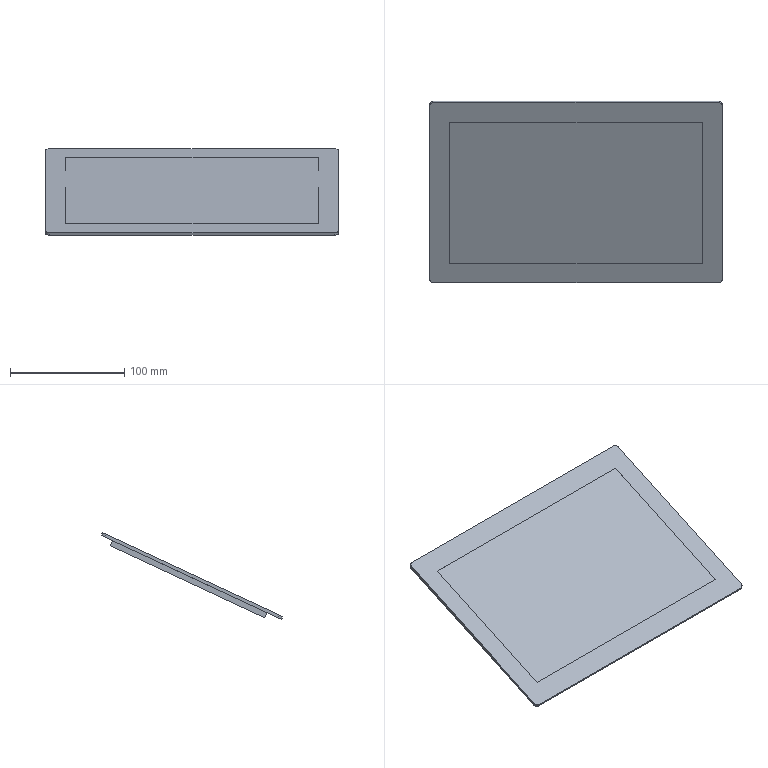Component | SolidWorks | 10.1InchScreen-1 | 1 solid | 20 faces | box 256.55 x 159.21 x 76.01 mm | volume 282503 mm3 | plane 16 | cylinder 4 | commonest cylinder face diameters 7 x4
build123d program:
from build123d import *

# Parameters (mm, degrees)
BOSS_EXTRUDE1_DEPTH = 2.5
SKETCH2_W           = 228.95
SKETCH2_H           = 149.3
BOSS_EXTRUDE2_DEPTH = 5
SKETCH3_W           = 221.1
SKETCH3_H           = 136.4
CUT_EXTRUDE1_DEPTH  = 0.01


with BuildPart() as part:
    # Sketch1 → Boss-Extrude1 (new body)
    with BuildSketch(Plane.XY):
        with BuildLine():
            Line((-124.775, -87.25), (124.775, -87.25))
            ThreePointArc((124.775, -87.25), (127.25, -86.225), (128.275, -83.75))
            Line((128.275, -83.75), (128.275, 83.75))
            ThreePointArc((128.275, 83.75), (127.25, 86.225), (124.775, 87.25))
            Line((124.775, 87.25), (-124.775, 87.25))
            ThreePointArc((-124.775, 87.25), (-127.25, 86.225), (-128.275, 83.75))
            Line((-128.275, 83.75), (-128.275, -83.75))
            ThreePointArc((-128.275, -83.75), (-127.25, -86.225), (-124.775, -87.25))
        make_face()
    extrude(amount=BOSS_EXTRUDE1_DEPTH)

    # Sketch2 → Boss-Extrude2 (add)
    with BuildSketch(Plane(origin=(0, 0, 0), x_dir=(-1, 0, 0), z_dir=(0, 0, -1))):
        with Locations((0, 1.4)):
            Rectangle(SKETCH2_W, SKETCH2_H)
    extrude(amount=BOSS_EXTRUDE2_DEPTH)

    # Sketch3 → Cut-Extrude1 (cut)
    with BuildSketch(Plane.XY.offset(2.5)):
        Rectangle(SKETCH3_W, SKETCH3_H)
    extrude(amount=-CUT_EXTRUDE1_DEPTH, mode=Mode.SUBTRACT)


solid = part.part

# Placed as in the assembly
solid = solid.moved(Location((1137.911, 1551.916, 2465.753), (25, 0, 0)))
STEP:
#1=CARTESIAN_POINT('',(49.712,57.986,95.625));
#2=VERTEX_POINT('',#1);
#3=CARTESIAN_POINT('',(49.85,58.111,95.683));
#4=VERTEX_POINT('',#3);
#5=CARTESIAN_POINT('',(49.712,58.111,95.683));
#6=DIRECTION('',(0.,-0.4226,0.9063));
#7=DIRECTION('',(1.,0.,0.));
#8=AXIS2_PLACEMENT_3D('',#5,#6,#7);
#9=CIRCLE('',#8,0.1378);
#10=EDGE_CURVE('',#2,#4,#9,.T.);
#11=ORIENTED_EDGE('',*,*,#10,.F.);
#12=CARTESIAN_POINT('',(39.887,57.986,95.625));
#13=VERTEX_POINT('',#12);
#14=CARTESIAN_POINT('',(39.887,57.986,95.625));
#15=DIRECTION('',(1.,0.,-0.));
#16=VECTOR('',#15,39.37);
#17=LINE('',#14,#16);
#18=EDGE_CURVE('',#13,#2,#17,.T.);
#19=ORIENTED_EDGE('',*,*,#18,.F.);
#20=CARTESIAN_POINT('',(39.749,58.111,95.683));
#21=VERTEX_POINT('',#20);
#22=CARTESIAN_POINT('',(39.887,58.111,95.683));
#23=DIRECTION('',(0.,-0.4226,0.9063));
#24=DIRECTION('',(-1.,0.,0.));
#25=AXIS2_PLACEMENT_3D('',#22,#23,#24);
#26=CIRCLE('',#25,0.1378);
#27=EDGE_CURVE('',#21,#13,#26,.T.);
#28=ORIENTED_EDGE('',*,*,#27,.F.);
#29=CARTESIAN_POINT('',(39.749,64.087,98.47));
#30=VERTEX_POINT('',#29);
#31=CARTESIAN_POINT('',(39.749,58.111,95.683));
#32=DIRECTION('',(-0.,-0.9063,-0.4226));
#33=VECTOR('',#32,39.37);
#34=LINE('',#31,#33);
#35=EDGE_CURVE('',#30,#21,#34,.T.);
#36=ORIENTED_EDGE('',*,*,#35,.F.);
#37=CARTESIAN_POINT('',(39.887,64.212,98.529));
#38=VERTEX_POINT('',#37);
#39=CARTESIAN_POINT('',(39.887,64.087,98.47));
#40=DIRECTION('',(0.,-0.4226,0.9063));
#41=DIRECTION('',(-1.,0.,0.));
#42=AXIS2_PLACEMENT_3D('',#39,#40,#41);
#43=CIRCLE('',#42,0.1378);
#44=EDGE_CURVE('',#38,#30,#43,.T.);
#45=ORIENTED_EDGE('',*,*,#44,.F.);
#46=CARTESIAN_POINT('',(49.712,64.212,98.529));
#47=VERTEX_POINT('',#46);
#48=CARTESIAN_POINT('',(39.887,64.212,98.529));
#49=DIRECTION('',(-1.,-0.,0.));
#50=VECTOR('',#49,39.37);
#51=LINE('',#48,#50);
#52=EDGE_CURVE('',#47,#38,#51,.T.);
#53=ORIENTED_EDGE('',*,*,#52,.F.);
#54=CARTESIAN_POINT('',(49.85,64.087,98.47));
#55=VERTEX_POINT('',#54);
#56=CARTESIAN_POINT('',(49.712,64.087,98.47));
#57=DIRECTION('',(0.,-0.4226,0.9063));
#58=DIRECTION('',(-1.,0.,0.));
#59=AXIS2_PLACEMENT_3D('',#56,#57,#58);
#60=CIRCLE('',#59,0.1378);
#61=EDGE_CURVE('',#55,#47,#60,.T.);
#62=ORIENTED_EDGE('',*,*,#61,.F.);
#63=CARTESIAN_POINT('',(49.85,58.111,95.683));
#64=DIRECTION('',(0.,0.9063,0.4226));
#65=VECTOR('',#64,39.37);
#66=LINE('',#63,#65);
#67=EDGE_CURVE('',#4,#55,#66,.T.);
#68=ORIENTED_EDGE('',*,*,#67,.F.);
#69=EDGE_LOOP('',(#11,#19,#28,#36,#45,#53,#62,#68));
#70=FACE_OUTER_BOUND('',#69,.T.);
#71=CARTESIAN_POINT('',(40.293,58.485,95.858));
#72=VERTEX_POINT('',#71);
#73=CARTESIAN_POINT('',(40.293,63.813,98.342));
#74=VERTEX_POINT('',#73);
#75=CARTESIAN_POINT('',(40.293,58.485,95.858));
#76=DIRECTION('',(0.,0.9063,0.4226));
#77=VECTOR('',#76,39.37);
#78=LINE('',#75,#77);
#79=EDGE_CURVE('',#72,#74,#78,.T.);
#80=ORIENTED_EDGE('',*,*,#79,.F.);
#81=CARTESIAN_POINT('',(49.307,58.485,95.858));
#82=VERTEX_POINT('',#81);
#83=CARTESIAN_POINT('',(49.307,58.485,95.858));
#84=DIRECTION('',(-1.,-0.,0.));
#85=VECTOR('',#84,39.37);
#86=LINE('',#83,#85);
#87=EDGE_CURVE('',#82,#72,#86,.T.);
#88=ORIENTED_EDGE('',*,*,#87,.F.);
#89=CARTESIAN_POINT('',(49.307,63.813,98.342));
#90=VERTEX_POINT('',#89);
#91=CARTESIAN_POINT('',(49.307,58.485,95.858));
#92=DIRECTION('',(-0.,-0.9063,-0.4226));
#93=VECTOR('',#92,39.37);
#94=LINE('',#91,#93);
#95=EDGE_CURVE('',#90,#82,#94,.T.);
#96=ORIENTED_EDGE('',*,*,#95,.F.);
#97=CARTESIAN_POINT('',(49.307,63.813,98.342));
#98=DIRECTION('',(1.,0.,-0.));
#99=VECTOR('',#98,39.37);
#100=LINE('',#97,#99);
#101=EDGE_CURVE('',#74,#90,#100,.T.);
#102=ORIENTED_EDGE('',*,*,#101,.F.);
#103=EDGE_LOOP('',(#80,#88,#96,#102));
#104=FACE_BOUND('',#103,.T.);
#105=CARTESIAN_POINT('',(49.712,58.111,95.683));
#106=DIRECTION('',(0.,-0.4226,0.9063));
#107=DIRECTION('',(1.,0.,-0.));
#108=AXIS2_PLACEMENT_3D('',#105,#106,#107);
#109=PLANE('',#108);
#110=ADVANCED_FACE('',(#70,#104),#109,.F.);
#111=ORIENTED_EDGE('',*,*,#10,.T.);
#112=CARTESIAN_POINT('',(49.85,58.069,95.773));
#113=VERTEX_POINT('',#112);
#114=CARTESIAN_POINT('',(49.85,58.069,95.773));
#115=DIRECTION('',(-0.,0.4226,-0.9063));
#116=VECTOR('',#115,39.37);
#117=LINE('',#114,#116);
#118=EDGE_CURVE('',#113,#4,#117,.T.);
#119=ORIENTED_EDGE('',*,*,#118,.F.);
#120=CARTESIAN_POINT('',(49.712,57.944,95.714));
#121=VERTEX_POINT('',#120);
#122=CARTESIAN_POINT('',(49.712,58.069,95.773));
#123=DIRECTION('',(0.,-0.4226,0.9063));
#124=DIRECTION('',(1.,0.,0.));
#125=AXIS2_PLACEMENT_3D('',#122,#123,#124);
#126=CIRCLE('',#125,0.1378);
#127=EDGE_CURVE('',#121,#113,#126,.T.);
#128=ORIENTED_EDGE('',*,*,#127,.F.);
#129=CARTESIAN_POINT('',(49.712,57.944,95.714));
#130=DIRECTION('',(-0.,0.4226,-0.9063));
#131=VECTOR('',#130,39.37);
#132=LINE('',#129,#131);
#133=EDGE_CURVE('',#121,#2,#132,.T.);
#134=ORIENTED_EDGE('',*,*,#133,.T.);
#135=EDGE_LOOP('',(#111,#119,#128,#134));
#136=FACE_OUTER_BOUND('',#135,.T.);
#137=CARTESIAN_POINT('',(49.712,58.069,95.773));
#138=DIRECTION('',(-0.,0.4226,-0.9063));
#139=DIRECTION('',(-1.,0.,0.));
#140=AXIS2_PLACEMENT_3D('',#137,#138,#139);
#141=CYLINDRICAL_SURFACE('',#140,0.1378);
#142=ADVANCED_FACE('',(#136),#141,.T.);
#143=ORIENTED_EDGE('',*,*,#67,.T.);
#144=CARTESIAN_POINT('',(49.85,64.046,98.56));
#145=VERTEX_POINT('',#144);
#146=CARTESIAN_POINT('',(49.85,64.046,98.56));
#147=DIRECTION('',(-0.,0.4226,-0.9063));
#148=VECTOR('',#147,39.37);
#149=LINE('',#146,#148);
#150=EDGE_CURVE('',#145,#55,#149,.T.);
#151=ORIENTED_EDGE('',*,*,#150,.F.);
#152=CARTESIAN_POINT('',(49.85,58.069,95.773));
#153=DIRECTION('',(0.,0.9063,0.4226));
#154=VECTOR('',#153,39.37);
#155=LINE('',#152,#154);
#156=EDGE_CURVE('',#113,#145,#155,.T.);
#157=ORIENTED_EDGE('',*,*,#156,.F.);
#158=ORIENTED_EDGE('',*,*,#118,.T.);
#159=EDGE_LOOP('',(#143,#151,#157,#158));
#160=FACE_OUTER_BOUND('',#159,.T.);
#161=CARTESIAN_POINT('',(49.85,58.069,95.773));
#162=DIRECTION('',(-1.,-0.,0.));
#163=DIRECTION('',(0.,-0.4226,0.9063));
#164=AXIS2_PLACEMENT_3D('',#161,#162,#163);
#165=PLANE('',#164);
#166=ADVANCED_FACE('',(#160),#165,.F.);
#167=ORIENTED_EDGE('',*,*,#61,.T.);
#168=CARTESIAN_POINT('',(49.712,64.171,98.618));
#169=VERTEX_POINT('',#168);
#170=CARTESIAN_POINT('',(49.712,64.171,98.618));
#171=DIRECTION('',(-0.,0.4226,-0.9063));
#172=VECTOR('',#171,39.37);
#173=LINE('',#170,#172);
#174=EDGE_CURVE('',#169,#47,#173,.T.);
#175=ORIENTED_EDGE('',*,*,#174,.F.);
#176=CARTESIAN_POINT('',(49.712,64.046,98.56));
#177=DIRECTION('',(0.,-0.4226,0.9063));
#178=DIRECTION('',(-1.,0.,0.));
#179=AXIS2_PLACEMENT_3D('',#176,#177,#178);
#180=CIRCLE('',#179,0.1378);
#181=EDGE_CURVE('',#145,#169,#180,.T.);
#182=ORIENTED_EDGE('',*,*,#181,.F.);
#183=ORIENTED_EDGE('',*,*,#150,.T.);
#184=EDGE_LOOP('',(#167,#175,#182,#183));
#185=FACE_OUTER_BOUND('',#184,.T.);
#186=CARTESIAN_POINT('',(49.712,64.046,98.56));
#187=DIRECTION('',(-0.,0.4226,-0.9063));
#188=DIRECTION('',(-1.,0.,0.));
#189=AXIS2_PLACEMENT_3D('',#186,#187,#188);
#190=CYLINDRICAL_SURFACE('',#189,0.1378);
#191=ADVANCED_FACE('',(#185),#190,.T.);
#192=ORIENTED_EDGE('',*,*,#52,.T.);
#193=CARTESIAN_POINT('',(39.887,64.171,98.618));
#194=VERTEX_POINT('',#193);
#195=CARTESIAN_POINT('',(39.887,64.171,98.618));
#196=DIRECTION('',(-0.,0.4226,-0.9063));
#197=VECTOR('',#196,39.37);
#198=LINE('',#195,#197);
#199=EDGE_CURVE('',#194,#38,#198,.T.);
#200=ORIENTED_EDGE('',*,*,#199,.F.);
#201=CARTESIAN_POINT('',(39.887,64.171,98.618));
#202=DIRECTION('',(-1.,-0.,0.));
#203=VECTOR('',#202,39.37);
#204=LINE('',#201,#203);
#205=EDGE_CURVE('',#169,#194,#204,.T.);
#206=ORIENTED_EDGE('',*,*,#205,.F.);
#207=ORIENTED_EDGE('',*,*,#174,.T.);
#208=EDGE_LOOP('',(#192,#200,#206,#207));
#209=FACE_OUTER_BOUND('',#208,.T.);
#210=CARTESIAN_POINT('',(39.887,64.171,98.618));
#211=DIRECTION('',(-0.,-0.9063,-0.4226));
#212=DIRECTION('',(-0.,0.4226,-0.9063));
#213=AXIS2_PLACEMENT_3D('',#210,#211,#212);
#214=PLANE('',#213);
#215=ADVANCED_FACE('',(#209),#214,.F.);
#216=ORIENTED_EDGE('',*,*,#44,.T.);
#217=CARTESIAN_POINT('',(39.749,64.046,98.56));
#218=VERTEX_POINT('',#217);
#219=CARTESIAN_POINT('',(39.749,64.046,98.56));
#220=DIRECTION('',(-0.,0.4226,-0.9063));
#221=VECTOR('',#220,39.37);
#222=LINE('',#219,#221);
#223=EDGE_CURVE('',#218,#30,#222,.T.);
#224=ORIENTED_EDGE('',*,*,#223,.F.);
#225=CARTESIAN_POINT('',(39.887,64.046,98.56));
#226=DIRECTION('',(0.,-0.4226,0.9063));
#227=DIRECTION('',(-1.,0.,0.));
#228=AXIS2_PLACEMENT_3D('',#225,#226,#227);
#229=CIRCLE('',#228,0.1378);
#230=EDGE_CURVE('',#194,#218,#229,.T.);
#231=ORIENTED_EDGE('',*,*,#230,.F.);
#232=ORIENTED_EDGE('',*,*,#199,.T.);
#233=EDGE_LOOP('',(#216,#224,#231,#232));
#234=FACE_OUTER_BOUND('',#233,.T.);
#235=CARTESIAN_POINT('',(39.887,64.046,98.56));
#236=DIRECTION('',(-0.,0.4226,-0.9063));
#237=DIRECTION('',(-1.,0.,0.));
#238=AXIS2_PLACEMENT_3D('',#235,#236,#237);
#239=CYLINDRICAL_SURFACE('',#238,0.1378);
#240=ADVANCED_FACE('',(#234),#239,.T.);
#241=ORIENTED_EDGE('',*,*,#35,.T.);
#242=CARTESIAN_POINT('',(39.749,58.069,95.773));
#243=VERTEX_POINT('',#242);
#244=CARTESIAN_POINT('',(39.749,58.069,95.773));
#245=DIRECTION('',(-0.,0.4226,-0.9063));
#246=VECTOR('',#245,39.37);
#247=LINE('',#244,#246);
#248=EDGE_CURVE('',#243,#21,#247,.T.);
#249=ORIENTED_EDGE('',*,*,#248,.F.);
#250=CARTESIAN_POINT('',(39.749,58.069,95.773));
#251=DIRECTION('',(-0.,-0.9063,-0.4226));
#252=VECTOR('',#251,39.37);
#253=LINE('',#250,#252);
#254=EDGE_CURVE('',#218,#243,#253,.T.);
#255=ORIENTED_EDGE('',*,*,#254,.F.);
#256=ORIENTED_EDGE('',*,*,#223,.T.);
#257=EDGE_LOOP('',(#241,#249,#255,#256));
#258=FACE_OUTER_BOUND('',#257,.T.);
#259=CARTESIAN_POINT('',(39.749,58.069,95.773));
#260=DIRECTION('',(1.,0.,-0.));
#261=DIRECTION('',(-0.,0.4226,-0.9063));
#262=AXIS2_PLACEMENT_3D('',#259,#260,#261);
#263=PLANE('',#262);
#264=ADVANCED_FACE('',(#258),#263,.F.);
#265=ORIENTED_EDGE('',*,*,#27,.T.);
#266=CARTESIAN_POINT('',(39.887,57.944,95.714));
#267=VERTEX_POINT('',#266);
#268=CARTESIAN_POINT('',(39.887,57.944,95.714));
#269=DIRECTION('',(-0.,0.4226,-0.9063));
#270=VECTOR('',#269,39.37);
#271=LINE('',#268,#270);
#272=EDGE_CURVE('',#267,#13,#271,.T.);
#273=ORIENTED_EDGE('',*,*,#272,.F.);
#274=CARTESIAN_POINT('',(39.887,58.069,95.773));
#275=DIRECTION('',(0.,-0.4226,0.9063));
#276=DIRECTION('',(-1.,0.,0.));
#277=AXIS2_PLACEMENT_3D('',#274,#275,#276);
#278=CIRCLE('',#277,0.1378);
#279=EDGE_CURVE('',#243,#267,#278,.T.);
#280=ORIENTED_EDGE('',*,*,#279,.F.);
#281=ORIENTED_EDGE('',*,*,#248,.T.);
#282=EDGE_LOOP('',(#265,#273,#280,#281));
#283=FACE_OUTER_BOUND('',#282,.T.);
#284=CARTESIAN_POINT('',(39.887,58.069,95.773));
#285=DIRECTION('',(-0.,0.4226,-0.9063));
#286=DIRECTION('',(-1.,0.,0.));
#287=AXIS2_PLACEMENT_3D('',#284,#285,#286);
#288=CYLINDRICAL_SURFACE('',#287,0.1378);
#289=ADVANCED_FACE('',(#283),#288,.T.);
#290=ORIENTED_EDGE('',*,*,#18,.T.);
#291=ORIENTED_EDGE('',*,*,#133,.F.);
#292=CARTESIAN_POINT('',(39.887,57.944,95.714));
#293=DIRECTION('',(1.,0.,-0.));
#294=VECTOR('',#293,39.37);
#295=LINE('',#292,#294);
#296=EDGE_CURVE('',#267,#121,#295,.T.);
#297=ORIENTED_EDGE('',*,*,#296,.F.);
#298=ORIENTED_EDGE('',*,*,#272,.T.);
#299=EDGE_LOOP('',(#290,#291,#297,#298));
#300=FACE_OUTER_BOUND('',#299,.T.);
#301=CARTESIAN_POINT('',(39.887,57.944,95.714));
#302=DIRECTION('',(0.,0.9063,0.4226));
#303=DIRECTION('',(0.,-0.4226,0.9063));
#304=AXIS2_PLACEMENT_3D('',#301,#302,#303);
#305=PLANE('',#304);
#306=ADVANCED_FACE('',(#300),#305,.F.);
#307=CARTESIAN_POINT('',(49.152,58.624,96.031));
#308=VERTEX_POINT('',#307);
#309=CARTESIAN_POINT('',(49.152,63.491,98.301));
#310=VERTEX_POINT('',#309);
#311=CARTESIAN_POINT('',(49.152,58.624,96.031));
#312=DIRECTION('',(0.,0.9063,0.4226));
#313=VECTOR('',#312,39.37);
#314=LINE('',#311,#313);
#315=EDGE_CURVE('',#308,#310,#314,.T.);
#316=ORIENTED_EDGE('',*,*,#315,.F.);
#317=CARTESIAN_POINT('',(40.447,58.624,96.031));
#318=VERTEX_POINT('',#317);
#319=CARTESIAN_POINT('',(40.447,58.624,96.031));
#320=DIRECTION('',(1.,0.,-0.));
#321=VECTOR('',#320,39.37);
#322=LINE('',#319,#321);
#323=EDGE_CURVE('',#318,#308,#322,.T.);
#324=ORIENTED_EDGE('',*,*,#323,.F.);
#325=CARTESIAN_POINT('',(40.447,63.491,98.301));
#326=VERTEX_POINT('',#325);
#327=CARTESIAN_POINT('',(40.447,58.624,96.031));
#328=DIRECTION('',(-0.,-0.9063,-0.4226));
#329=VECTOR('',#328,39.37);
#330=LINE('',#327,#329);
#331=EDGE_CURVE('',#326,#318,#330,.T.);
#332=ORIENTED_EDGE('',*,*,#331,.F.);
#333=CARTESIAN_POINT('',(40.447,63.491,98.301));
#334=DIRECTION('',(-1.,-0.,0.));
#335=VECTOR('',#334,39.37);
#336=LINE('',#333,#335);
#337=EDGE_CURVE('',#310,#326,#336,.T.);
#338=ORIENTED_EDGE('',*,*,#337,.F.);
#339=EDGE_LOOP('',(#316,#324,#332,#338));
#340=FACE_BOUND('',#339,.T.);
#341=ORIENTED_EDGE('',*,*,#127,.T.);
#342=ORIENTED_EDGE('',*,*,#156,.T.);
#343=ORIENTED_EDGE('',*,*,#181,.T.);
#344=ORIENTED_EDGE('',*,*,#205,.T.);
#345=ORIENTED_EDGE('',*,*,#230,.T.);
#346=ORIENTED_EDGE('',*,*,#254,.T.);
#347=ORIENTED_EDGE('',*,*,#279,.T.);
#348=ORIENTED_EDGE('',*,*,#296,.T.);
#349=EDGE_LOOP('',(#341,#342,#343,#344,#345,#346,#347,#348));
#350=FACE_OUTER_BOUND('',#349,.T.);
#351=CARTESIAN_POINT('',(49.712,58.069,95.773));
#352=DIRECTION('',(0.,-0.4226,0.9063));
#353=DIRECTION('',(1.,0.,-0.));
#354=AXIS2_PLACEMENT_3D('',#351,#352,#353);
#355=PLANE('',#354);
#356=ADVANCED_FACE('',(#340,#350),#355,.T.);
#357=ORIENTED_EDGE('',*,*,#79,.T.);
#358=CARTESIAN_POINT('',(40.293,63.896,98.164));
#359=VERTEX_POINT('',#358);
#360=CARTESIAN_POINT('',(40.293,63.896,98.164));
#361=DIRECTION('',(0.,-0.4226,0.9063));
#362=VECTOR('',#361,39.37);
#363=LINE('',#360,#362);
#364=EDGE_CURVE('',#359,#74,#363,.T.);
#365=ORIENTED_EDGE('',*,*,#364,.F.);
#366=CARTESIAN_POINT('',(40.293,58.569,95.68));
#367=VERTEX_POINT('',#366);
#368=CARTESIAN_POINT('',(40.293,58.569,95.68));
#369=DIRECTION('',(0.,0.9063,0.4226));
#370=VECTOR('',#369,39.37);
#371=LINE('',#368,#370);
#372=EDGE_CURVE('',#367,#359,#371,.T.);
#373=ORIENTED_EDGE('',*,*,#372,.F.);
#374=CARTESIAN_POINT('',(40.293,58.569,95.68));
#375=DIRECTION('',(0.,-0.4226,0.9063));
#376=VECTOR('',#375,39.37);
#377=LINE('',#374,#376);
#378=EDGE_CURVE('',#367,#72,#377,.T.);
#379=ORIENTED_EDGE('',*,*,#378,.T.);
#380=EDGE_LOOP('',(#357,#365,#373,#379));
#381=FACE_OUTER_BOUND('',#380,.T.);
#382=CARTESIAN_POINT('',(40.293,58.569,95.68));
#383=DIRECTION('',(1.,0.,-0.));
#384=DIRECTION('',(-0.,0.4226,-0.9063));
#385=AXIS2_PLACEMENT_3D('',#382,#383,#384);
#386=PLANE('',#385);
#387=ADVANCED_FACE('',(#381),#386,.F.);
#388=ORIENTED_EDGE('',*,*,#101,.T.);
#389=CARTESIAN_POINT('',(49.307,63.896,98.164));
#390=VERTEX_POINT('',#389);
#391=CARTESIAN_POINT('',(49.307,63.896,98.164));
#392=DIRECTION('',(0.,-0.4226,0.9063));
#393=VECTOR('',#392,39.37);
#394=LINE('',#391,#393);
#395=EDGE_CURVE('',#390,#90,#394,.T.);
#396=ORIENTED_EDGE('',*,*,#395,.F.);
#397=CARTESIAN_POINT('',(49.307,63.896,98.164));
#398=DIRECTION('',(1.,0.,-0.));
#399=VECTOR('',#398,39.37);
#400=LINE('',#397,#399);
#401=EDGE_CURVE('',#359,#390,#400,.T.);
#402=ORIENTED_EDGE('',*,*,#401,.F.);
#403=ORIENTED_EDGE('',*,*,#364,.T.);
#404=EDGE_LOOP('',(#388,#396,#402,#403));
#405=FACE_OUTER_BOUND('',#404,.T.);
#406=CARTESIAN_POINT('',(49.307,63.896,98.164));
#407=DIRECTION('',(-0.,-0.9063,-0.4226));
#408=DIRECTION('',(-0.,0.4226,-0.9063));
#409=AXIS2_PLACEMENT_3D('',#406,#407,#408);
#410=PLANE('',#409);
#411=ADVANCED_FACE('',(#405),#410,.F.);
#412=ORIENTED_EDGE('',*,*,#95,.T.);
#413=CARTESIAN_POINT('',(49.307,58.569,95.68));
#414=VERTEX_POINT('',#413);
#415=CARTESIAN_POINT('',(49.307,58.569,95.68));
#416=DIRECTION('',(0.,-0.4226,0.9063));
#417=VECTOR('',#416,39.37);
#418=LINE('',#415,#417);
#419=EDGE_CURVE('',#414,#82,#418,.T.);
#420=ORIENTED_EDGE('',*,*,#419,.F.);
#421=CARTESIAN_POINT('',(49.307,58.569,95.68));
#422=DIRECTION('',(-0.,-0.9063,-0.4226));
#423=VECTOR('',#422,39.37);
#424=LINE('',#421,#423);
#425=EDGE_CURVE('',#390,#414,#424,.T.);
#426=ORIENTED_EDGE('',*,*,#425,.F.);
#427=ORIENTED_EDGE('',*,*,#395,.T.);
#428=EDGE_LOOP('',(#412,#420,#426,#427));
#429=FACE_OUTER_BOUND('',#428,.T.);
#430=CARTESIAN_POINT('',(49.307,58.569,95.68));
#431=DIRECTION('',(-1.,-0.,0.));
#432=DIRECTION('',(0.,-0.4226,0.9063));
#433=AXIS2_PLACEMENT_3D('',#430,#431,#432);
#434=PLANE('',#433);
#435=ADVANCED_FACE('',(#429),#434,.F.);
#436=ORIENTED_EDGE('',*,*,#87,.T.);
#437=ORIENTED_EDGE('',*,*,#378,.F.);
#438=CARTESIAN_POINT('',(49.307,58.569,95.68));
#439=DIRECTION('',(-1.,-0.,0.));
#440=VECTOR('',#439,39.37);
#441=LINE('',#438,#440);
#442=EDGE_CURVE('',#414,#367,#441,.T.);
#443=ORIENTED_EDGE('',*,*,#442,.F.);
#444=ORIENTED_EDGE('',*,*,#419,.T.);
#445=EDGE_LOOP('',(#436,#437,#443,#444));
#446=FACE_OUTER_BOUND('',#445,.T.);
#447=CARTESIAN_POINT('',(49.307,58.569,95.68));
#448=DIRECTION('',(0.,0.9063,0.4226));
#449=DIRECTION('',(0.,-0.4226,0.9063));
#450=AXIS2_PLACEMENT_3D('',#447,#448,#449);
#451=PLANE('',#450);
#452=ADVANCED_FACE('',(#446),#451,.F.);
#453=ORIENTED_EDGE('',*,*,#372,.T.);
#454=ORIENTED_EDGE('',*,*,#401,.T.);
#455=ORIENTED_EDGE('',*,*,#425,.T.);
#456=ORIENTED_EDGE('',*,*,#442,.T.);
#457=EDGE_LOOP('',(#453,#454,#455,#456));
#458=FACE_OUTER_BOUND('',#457,.T.);
#459=CARTESIAN_POINT('',(44.8,61.182,96.898));
#460=DIRECTION('',(0.,-0.4226,0.9063));
#461=DIRECTION('',(1.,0.,-0.));
#462=AXIS2_PLACEMENT_3D('',#459,#460,#461);
#463=PLANE('',#462);
#464=ADVANCED_FACE('',(#458),#463,.F.);
#465=ORIENTED_EDGE('',*,*,#315,.T.);
#466=CARTESIAN_POINT('',(49.152,63.491,98.3));
#467=VERTEX_POINT('',#466);
#468=CARTESIAN_POINT('',(49.152,63.491,98.3));
#469=DIRECTION('',(0.,-0.4226,0.9063));
#470=VECTOR('',#469,39.37);
#471=LINE('',#468,#470);
#472=EDGE_CURVE('',#467,#310,#471,.T.);
#473=ORIENTED_EDGE('',*,*,#472,.F.);
#474=CARTESIAN_POINT('',(49.152,58.624,96.031));
#475=VERTEX_POINT('',#474);
#476=CARTESIAN_POINT('',(49.152,58.624,96.031));
#477=DIRECTION('',(0.,0.9063,0.4226));
#478=VECTOR('',#477,39.37);
#479=LINE('',#476,#478);
#480=EDGE_CURVE('',#475,#467,#479,.T.);
#481=ORIENTED_EDGE('',*,*,#480,.F.);
#482=CARTESIAN_POINT('',(49.152,58.624,96.031));
#483=DIRECTION('',(0.,-0.4226,0.9063));
#484=VECTOR('',#483,39.37);
#485=LINE('',#482,#484);
#486=EDGE_CURVE('',#475,#308,#485,.T.);
#487=ORIENTED_EDGE('',*,*,#486,.T.);
#488=EDGE_LOOP('',(#465,#473,#481,#487));
#489=FACE_OUTER_BOUND('',#488,.T.);
#490=CARTESIAN_POINT('',(49.152,58.624,96.031));
#491=DIRECTION('',(1.,0.,-0.));
#492=DIRECTION('',(-0.,0.4226,-0.9063));
#493=AXIS2_PLACEMENT_3D('',#490,#491,#492);
#494=PLANE('',#493);
#495=ADVANCED_FACE('',(#489),#494,.F.);
#496=ORIENTED_EDGE('',*,*,#323,.T.);
#497=ORIENTED_EDGE('',*,*,#486,.F.);
#498=CARTESIAN_POINT('',(40.447,58.624,96.031));
#499=VERTEX_POINT('',#498);
#500=CARTESIAN_POINT('',(40.447,58.624,96.031));
#501=DIRECTION('',(1.,0.,-0.));
#502=VECTOR('',#501,39.37);
#503=LINE('',#500,#502);
#504=EDGE_CURVE('',#499,#475,#503,.T.);
#505=ORIENTED_EDGE('',*,*,#504,.F.);
#506=CARTESIAN_POINT('',(40.447,58.624,96.031));
#507=DIRECTION('',(0.,-0.4226,0.9063));
#508=VECTOR('',#507,39.37);
#509=LINE('',#506,#508);
#510=EDGE_CURVE('',#499,#318,#509,.T.);
#511=ORIENTED_EDGE('',*,*,#510,.T.);
#512=EDGE_LOOP('',(#496,#497,#505,#511));
#513=FACE_OUTER_BOUND('',#512,.T.);
#514=CARTESIAN_POINT('',(40.447,58.624,96.031));
#515=DIRECTION('',(-0.,-0.9063,-0.4226));
#516=DIRECTION('',(-0.,0.4226,-0.9063));
#517=AXIS2_PLACEMENT_3D('',#514,#515,#516);
#518=PLANE('',#517);
#519=ADVANCED_FACE('',(#513),#518,.F.);
#520=ORIENTED_EDGE('',*,*,#331,.T.);
#521=ORIENTED_EDGE('',*,*,#510,.F.);
#522=CARTESIAN_POINT('',(40.447,63.491,98.3));
#523=VERTEX_POINT('',#522);
#524=CARTESIAN_POINT('',(40.447,58.624,96.031));
#525=DIRECTION('',(-0.,-0.9063,-0.4226));
#526=VECTOR('',#525,39.37);
#527=LINE('',#524,#526);
#528=EDGE_CURVE('',#523,#499,#527,.T.);
#529=ORIENTED_EDGE('',*,*,#528,.F.);
#530=CARTESIAN_POINT('',(40.447,63.491,98.3));
#531=DIRECTION('',(0.,-0.4226,0.9063));
#532=VECTOR('',#531,39.37);
#533=LINE('',#530,#532);
#534=EDGE_CURVE('',#523,#326,#533,.T.);
#535=ORIENTED_EDGE('',*,*,#534,.T.);
#536=EDGE_LOOP('',(#520,#521,#529,#535));
#537=FACE_OUTER_BOUND('',#536,.T.);
#538=CARTESIAN_POINT('',(40.447,58.624,96.031));
#539=DIRECTION('',(-1.,-0.,0.));
#540=DIRECTION('',(0.,-0.4226,0.9063));
#541=AXIS2_PLACEMENT_3D('',#538,#539,#540);
#542=PLANE('',#541);
#543=ADVANCED_FACE('',(#537),#542,.F.);
#544=ORIENTED_EDGE('',*,*,#337,.T.);
#545=ORIENTED_EDGE('',*,*,#534,.F.);
#546=CARTESIAN_POINT('',(40.447,63.491,98.3));
#547=DIRECTION('',(-1.,-0.,0.));
#548=VECTOR('',#547,39.37);
#549=LINE('',#546,#548);
#550=EDGE_CURVE('',#467,#523,#549,.T.);
#551=ORIENTED_EDGE('',*,*,#550,.F.);
#552=ORIENTED_EDGE('',*,*,#472,.T.);
#553=EDGE_LOOP('',(#544,#545,#551,#552));
#554=FACE_OUTER_BOUND('',#553,.T.);
#555=CARTESIAN_POINT('',(40.447,63.491,98.3));
#556=DIRECTION('',(0.,0.9063,0.4226));
#557=DIRECTION('',(0.,-0.4226,0.9063));
#558=AXIS2_PLACEMENT_3D('',#555,#556,#557);
#559=PLANE('',#558);
#560=ADVANCED_FACE('',(#554),#559,.F.);
#561=ORIENTED_EDGE('',*,*,#480,.T.);
#562=ORIENTED_EDGE('',*,*,#550,.T.);
#563=ORIENTED_EDGE('',*,*,#528,.T.);
#564=ORIENTED_EDGE('',*,*,#504,.T.);
#565=EDGE_LOOP('',(#561,#562,#563,#564));
#566=FACE_OUTER_BOUND('',#565,.T.);
#567=CARTESIAN_POINT('',(44.8,61.058,97.166));
#568=DIRECTION('',(-0.,0.4226,-0.9063));
#569=DIRECTION('',(-1.,-0.,0.));
#570=AXIS2_PLACEMENT_3D('',#567,#568,#569);
#571=PLANE('',#570);
#572=ADVANCED_FACE('',(#566),#571,.F.);
#573=CLOSED_SHELL('',(#110,#142,#166,#191,#215,#240,#264,#289,#306,#356,#387,#411,#435,#452,#464,#495,#519,#543,#560,#572));
#574=MANIFOLD_SOLID_BREP('',#573);
#575=CARTESIAN_POINT('',(0.,0.,0.));
#576=DIRECTION('',(0.,0.,1.));
#577=DIRECTION('',(1.,0.,0.));
#578=AXIS2_PLACEMENT_3D('',#575,#576,#577);
#579=(LENGTH_UNIT()NAMED_UNIT(*)SI_UNIT($,.METRE.));
#580=LENGTH_MEASURE_WITH_UNIT(LENGTH_MEASURE(0.0254),#579);
#581=DIMENSIONAL_EXPONENTS(1.,0.,0.,0.,0.,0.,0.);
#582=(CONVERSION_BASED_UNIT('',#580)LENGTH_UNIT()NAMED_UNIT(#581));
#583=UNCERTAINTY_MEASURE_WITH_UNIT(LENGTH_MEASURE(0.00001),#582,'','');
#584=(NAMED_UNIT(*)PLANE_ANGLE_UNIT()SI_UNIT($,.RADIAN.));
#585=(NAMED_UNIT(*)SI_UNIT($,.STERADIAN.)SOLID_ANGLE_UNIT());
#586=(GEOMETRIC_REPRESENTATION_CONTEXT(3)GLOBAL_UNCERTAINTY_ASSIGNED_CONTEXT((#583))GLOBAL_UNIT_ASSIGNED_CONTEXT((#582,#584,#585))REPRESENTATION_CONTEXT('',''));
#587=ADVANCED_BREP_SHAPE_REPRESENTATION('',(#574,#578),#586);
#588=COLOUR_RGB('',0.7922,0.8196,0.9333);
#589=FILL_AREA_STYLE_COLOUR('',#588);
#590=FILL_AREA_STYLE('',(#589));
#591=SURFACE_STYLE_FILL_AREA(#590);
#592=SURFACE_SIDE_STYLE('',(#591));
#593=SURFACE_STYLE_USAGE(.BOTH.,#592);
#594=PRESENTATION_STYLE_ASSIGNMENT((#593));
#595=STYLED_ITEM('',(#594),#574);
#596=(LENGTH_UNIT()NAMED_UNIT(*)SI_UNIT($,.METRE.));
#597=LENGTH_MEASURE_WITH_UNIT(LENGTH_MEASURE(0.0254),#596);
#598=DIMENSIONAL_EXPONENTS(1.,0.,0.,0.,0.,0.,0.);
#599=(CONVERSION_BASED_UNIT('',#597)LENGTH_UNIT()NAMED_UNIT(#598));
#600=UNCERTAINTY_MEASURE_WITH_UNIT(LENGTH_MEASURE(0.00001),#599,'','');
#601=(NAMED_UNIT(*)PLANE_ANGLE_UNIT()SI_UNIT($,.RADIAN.));
#602=(NAMED_UNIT(*)SI_UNIT($,.STERADIAN.)SOLID_ANGLE_UNIT());
#603=(GEOMETRIC_REPRESENTATION_CONTEXT(3)GLOBAL_UNCERTAINTY_ASSIGNED_CONTEXT((#600))GLOBAL_UNIT_ASSIGNED_CONTEXT((#599,#601,#602))REPRESENTATION_CONTEXT('',''));
#604=MECHANICAL_DESIGN_GEOMETRIC_PRESENTATION_REPRESENTATION('',(#595),#603);
#605=PRESENTATION_LAYER_ASSIGNMENT('','',(#595));